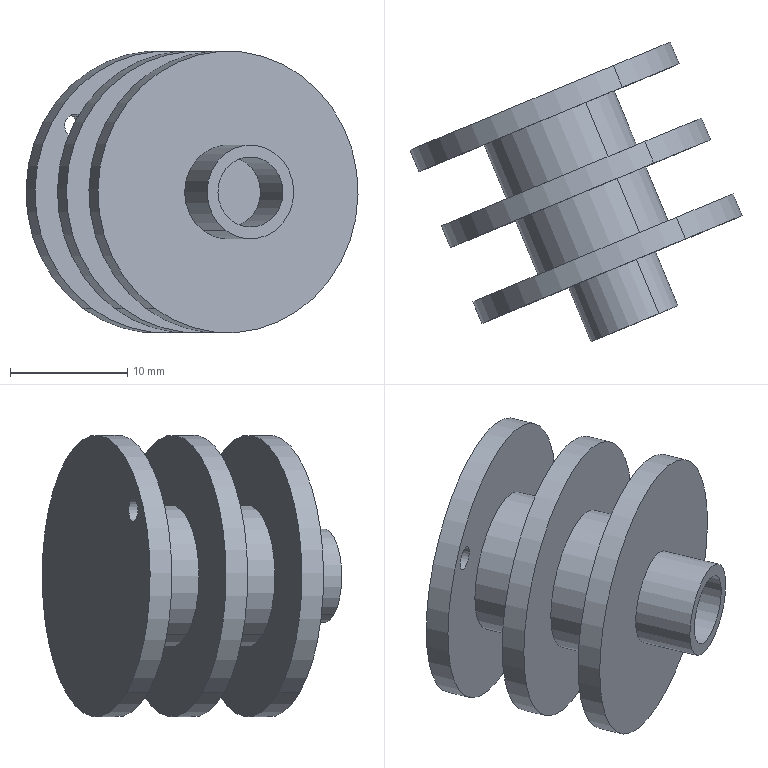Component | SolidWorks | Sensor-1 | 1 solid | 24 faces | box 28.3 x 25.53 x 24 mm | volume 3949 mm3 | cylinder 16 | plane 8 | commonest cylinder face diameters 24 x6 12 x4 2 x2 6 x2 8 x2
build123d program:
from build123d import *

# Parameters (mm, degrees)
SKETCH1_R           = 4
SKETCH1_R_2         = 3
BOSS_EXTRUDE1_DEPTH = 5
SKETCH2_R           = 12
BOSS_EXTRUDE2_DEPTH = 2
SKETCH3_R           = 6
BOSS_EXTRUDE3_DEPTH = 5
SKETCH4_R           = 12
BOSS_EXTRUDE4_DEPTH = 2
SKETCH5_R           = 6
BOSS_EXTRUDE5_DEPTH = 5
SKETCH6_R           = 12
BOSS_EXTRUDE6_DEPTH = 2
SKETCH7_R           = 1
CUT_EXTRUDE1_DEPTH  = 2


with BuildPart() as part:
    # Sketch1 → Boss-Extrude1 (new body)
    with BuildSketch(Plane.XY):
        Circle(SKETCH1_R)
        Circle(SKETCH1_R_2, mode=Mode.SUBTRACT)
    extrude(amount=BOSS_EXTRUDE1_DEPTH)

    # Sketch2 → Boss-Extrude2 (add)
    with BuildSketch(Plane.XY.offset(5)):
        Circle(SKETCH2_R)
    extrude(amount=BOSS_EXTRUDE2_DEPTH)

    # Sketch3 → Boss-Extrude3 (add)
    with BuildSketch(Plane.XY.offset(7)):
        Circle(SKETCH3_R)
    extrude(amount=BOSS_EXTRUDE3_DEPTH)

    # Sketch4 → Boss-Extrude4 (add)
    with BuildSketch(Plane.XY.offset(12)):
        Circle(SKETCH4_R)
    extrude(amount=BOSS_EXTRUDE4_DEPTH)

    # Sketch5 → Boss-Extrude5 (add)
    with BuildSketch(Plane.XY.offset(14)):
        Circle(SKETCH5_R)
    extrude(amount=BOSS_EXTRUDE5_DEPTH)

    # Sketch6 → Boss-Extrude6 (add)
    with BuildSketch(Plane.XY.offset(19)):
        Circle(SKETCH6_R)
    extrude(amount=BOSS_EXTRUDE6_DEPTH)

    # Sketch7 → Cut-Extrude1 (cut)
    with BuildSketch(Plane.XY.offset(21)):
        with Locations((0, 10)):
            Circle(SKETCH7_R)
    extrude(amount=-CUT_EXTRUDE1_DEPTH, mode=Mode.SUBTRACT)


solid = part.part

# Placed as in the assembly
solid = solid.moved(Location((25.514, 19.993, 407.896), (-90, -22.523, 124.32)))
STEP:
#1=COLOUR_RGB('',0.7922,0.8196,0.9333);
#2=FILL_AREA_STYLE_COLOUR('',#1);
#3=FILL_AREA_STYLE('',(#2));
#4=SURFACE_STYLE_FILL_AREA(#3);
#5=SURFACE_SIDE_STYLE('',(#4));
#6=SURFACE_STYLE_USAGE(.BOTH.,#5);
#7=PRESENTATION_STYLE_ASSIGNMENT((#6));
#8=CARTESIAN_POINT('',(0.4381,1.362,16.313));
#9=VERTEX_POINT('',#8);
#10=CARTESIAN_POINT('',(0.3971,1.345,16.248));
#11=VERTEX_POINT('',#10);
#12=CARTESIAN_POINT('',(0.4176,1.354,16.281));
#13=DIRECTION('',(-0.383,0.9237,-0.));
#14=DIRECTION('',(-0.5208,-0.216,-0.8259));
#15=AXIS2_PLACEMENT_3D('',#12,#13,#14);
#16=CIRCLE('',#15,0.03937);
#17=EDGE_CURVE('',#9,#11,#16,.T.);
#18=ORIENTED_EDGE('',*,*,#17,.F.);
#19=CARTESIAN_POINT('',(0.4079,1.435,16.313));
#20=VERTEX_POINT('',#19);
#21=CARTESIAN_POINT('',(0.4381,1.362,16.313));
#22=DIRECTION('',(-0.383,0.9237,-0.));
#23=VECTOR('',#22,39.37);
#24=LINE('',#21,#23);
#25=EDGE_CURVE('',#9,#20,#24,.T.);
#26=ORIENTED_EDGE('',*,*,#25,.T.);
#27=CARTESIAN_POINT('',(0.3669,1.418,16.248));
#28=VERTEX_POINT('',#27);
#29=CARTESIAN_POINT('',(0.3874,1.426,16.281));
#30=DIRECTION('',(-0.383,0.9237,-0.));
#31=DIRECTION('',(-0.5208,-0.216,-0.8259));
#32=AXIS2_PLACEMENT_3D('',#29,#30,#31);
#33=CIRCLE('',#32,0.03937);
#34=EDGE_CURVE('',#20,#28,#33,.T.);
#35=ORIENTED_EDGE('',*,*,#34,.T.);
#36=CARTESIAN_POINT('',(0.3971,1.345,16.248));
#37=DIRECTION('',(-0.383,0.9237,-0.));
#38=VECTOR('',#37,39.37);
#39=LINE('',#36,#38);
#40=EDGE_CURVE('',#11,#28,#39,.T.);
#41=ORIENTED_EDGE('',*,*,#40,.F.);
#42=EDGE_LOOP('',(#18,#26,#35,#41));
#43=FACE_OUTER_BOUND('',#42,.T.);
#44=CARTESIAN_POINT('',(0.4176,1.354,16.281));
#45=DIRECTION('',(-0.383,0.9237,-0.));
#46=DIRECTION('',(-0.5208,-0.216,-0.8259));
#47=AXIS2_PLACEMENT_3D('',#44,#45,#46);
#48=CYLINDRICAL_SURFACE('',#47,0.03937);
#49=ADVANCED_FACE('',(#43),#48,.F.);
#50=CARTESIAN_POINT('',(0.4417,1.449,15.669));
#51=VERTEX_POINT('',#50);
#52=CARTESIAN_POINT('',(0.9338,1.653,16.449));
#53=VERTEX_POINT('',#52);
#54=CARTESIAN_POINT('',(0.6878,1.551,16.059));
#55=DIRECTION('',(-0.383,0.9237,-0.));
#56=DIRECTION('',(-0.5208,-0.216,-0.8259));
#57=AXIS2_PLACEMENT_3D('',#54,#55,#56);
#58=CIRCLE('',#57,0.4724);
#59=EDGE_CURVE('',#51,#53,#58,.T.);
#60=ORIENTED_EDGE('',*,*,#59,.F.);
#61=CARTESIAN_POINT('',(0.4719,1.376,15.669));
#62=VERTEX_POINT('',#61);
#63=CARTESIAN_POINT('',(0.4417,1.449,15.669));
#64=DIRECTION('',(0.383,-0.9237,0.));
#65=VECTOR('',#64,39.37);
#66=LINE('',#63,#65);
#67=EDGE_CURVE('',#51,#62,#66,.T.);
#68=ORIENTED_EDGE('',*,*,#67,.T.);
#69=CARTESIAN_POINT('',(0.964,1.58,16.449));
#70=VERTEX_POINT('',#69);
#71=CARTESIAN_POINT('',(0.7179,1.478,16.059));
#72=DIRECTION('',(-0.383,0.9237,-0.));
#73=DIRECTION('',(-0.5208,-0.216,-0.8259));
#74=AXIS2_PLACEMENT_3D('',#71,#72,#73);
#75=CIRCLE('',#74,0.4724);
#76=EDGE_CURVE('',#62,#70,#75,.T.);
#77=ORIENTED_EDGE('',*,*,#76,.T.);
#78=CARTESIAN_POINT('',(0.9338,1.653,16.449));
#79=DIRECTION('',(0.383,-0.9237,0.));
#80=VECTOR('',#79,39.37);
#81=LINE('',#78,#80);
#82=EDGE_CURVE('',#53,#70,#81,.T.);
#83=ORIENTED_EDGE('',*,*,#82,.F.);
#84=EDGE_LOOP('',(#60,#68,#77,#83));
#85=FACE_OUTER_BOUND('',#84,.T.);
#86=CARTESIAN_POINT('',(0.6878,1.551,16.059));
#87=DIRECTION('',(0.383,-0.9237,0.));
#88=DIRECTION('',(0.5208,0.216,0.8259));
#89=AXIS2_PLACEMENT_3D('',#86,#87,#88);
#90=CYLINDRICAL_SURFACE('',#89,0.4724);
#91=ADVANCED_FACE('',(#85),#90,.T.);
#92=CARTESIAN_POINT('',(0.5949,1.427,15.864));
#93=VERTEX_POINT('',#92);
#94=CARTESIAN_POINT('',(0.841,1.529,16.254));
#95=VERTEX_POINT('',#94);
#96=CARTESIAN_POINT('',(0.7179,1.478,16.059));
#97=DIRECTION('',(-0.383,0.9237,-0.));
#98=DIRECTION('',(-0.5208,-0.216,-0.8259));
#99=AXIS2_PLACEMENT_3D('',#96,#97,#98);
#100=CIRCLE('',#99,0.2362);
#101=EDGE_CURVE('',#93,#95,#100,.T.);
#102=ORIENTED_EDGE('',*,*,#101,.F.);
#103=CARTESIAN_POINT('',(0.6703,1.245,15.864));
#104=VERTEX_POINT('',#103);
#105=CARTESIAN_POINT('',(0.5949,1.427,15.864));
#106=DIRECTION('',(0.383,-0.9237,0.));
#107=VECTOR('',#106,39.37);
#108=LINE('',#105,#107);
#109=EDGE_CURVE('',#93,#104,#108,.T.);
#110=ORIENTED_EDGE('',*,*,#109,.T.);
#111=CARTESIAN_POINT('',(0.9164,1.347,16.254));
#112=VERTEX_POINT('',#111);
#113=CARTESIAN_POINT('',(0.7933,1.296,16.059));
#114=DIRECTION('',(-0.383,0.9237,-0.));
#115=DIRECTION('',(-0.5208,-0.216,-0.8259));
#116=AXIS2_PLACEMENT_3D('',#113,#114,#115);
#117=CIRCLE('',#116,0.2362);
#118=EDGE_CURVE('',#104,#112,#117,.T.);
#119=ORIENTED_EDGE('',*,*,#118,.T.);
#120=CARTESIAN_POINT('',(0.841,1.529,16.254));
#121=DIRECTION('',(0.383,-0.9237,0.));
#122=VECTOR('',#121,39.37);
#123=LINE('',#120,#122);
#124=EDGE_CURVE('',#95,#112,#123,.T.);
#125=ORIENTED_EDGE('',*,*,#124,.F.);
#126=EDGE_LOOP('',(#102,#110,#119,#125));
#127=FACE_OUTER_BOUND('',#126,.T.);
#128=CARTESIAN_POINT('',(0.7179,1.478,16.059));
#129=DIRECTION('',(0.383,-0.9237,0.));
#130=DIRECTION('',(0.5208,0.216,0.8259));
#131=AXIS2_PLACEMENT_3D('',#128,#129,#130);
#132=CYLINDRICAL_SURFACE('',#131,0.2362);
#133=ADVANCED_FACE('',(#127),#132,.T.);
#134=CARTESIAN_POINT('',(0.5473,1.194,15.669));
#135=VERTEX_POINT('',#134);
#136=CARTESIAN_POINT('',(1.039,1.398,16.449));
#137=VERTEX_POINT('',#136);
#138=CARTESIAN_POINT('',(0.7933,1.296,16.059));
#139=DIRECTION('',(-0.383,0.9237,-0.));
#140=DIRECTION('',(-0.5208,-0.216,-0.8259));
#141=AXIS2_PLACEMENT_3D('',#138,#139,#140);
#142=CIRCLE('',#141,0.4724);
#143=EDGE_CURVE('',#135,#137,#142,.T.);
#144=ORIENTED_EDGE('',*,*,#143,.F.);
#145=CARTESIAN_POINT('',(0.5775,1.121,15.669));
#146=VERTEX_POINT('',#145);
#147=CARTESIAN_POINT('',(0.5473,1.194,15.669));
#148=DIRECTION('',(0.383,-0.9237,0.));
#149=VECTOR('',#148,39.37);
#150=LINE('',#147,#149);
#151=EDGE_CURVE('',#135,#146,#150,.T.);
#152=ORIENTED_EDGE('',*,*,#151,.T.);
#153=CARTESIAN_POINT('',(1.07,1.326,16.449));
#154=VERTEX_POINT('',#153);
#155=CARTESIAN_POINT('',(0.8235,1.224,16.059));
#156=DIRECTION('',(-0.383,0.9237,-0.));
#157=DIRECTION('',(-0.5208,-0.216,-0.8259));
#158=AXIS2_PLACEMENT_3D('',#155,#156,#157);
#159=CIRCLE('',#158,0.4724);
#160=EDGE_CURVE('',#146,#154,#159,.T.);
#161=ORIENTED_EDGE('',*,*,#160,.T.);
#162=CARTESIAN_POINT('',(1.039,1.398,16.449));
#163=DIRECTION('',(0.383,-0.9237,0.));
#164=VECTOR('',#163,39.37);
#165=LINE('',#162,#164);
#166=EDGE_CURVE('',#137,#154,#165,.T.);
#167=ORIENTED_EDGE('',*,*,#166,.F.);
#168=EDGE_LOOP('',(#144,#152,#161,#167));
#169=FACE_OUTER_BOUND('',#168,.T.);
#170=CARTESIAN_POINT('',(0.7933,1.296,16.059));
#171=DIRECTION('',(0.383,-0.9237,0.));
#172=DIRECTION('',(0.5208,0.216,0.8259));
#173=AXIS2_PLACEMENT_3D('',#170,#171,#172);
#174=CYLINDRICAL_SURFACE('',#173,0.4724);
#175=ADVANCED_FACE('',(#169),#174,.T.);
#176=CARTESIAN_POINT('',(0.7005,1.173,15.864));
#177=VERTEX_POINT('',#176);
#178=CARTESIAN_POINT('',(0.9465,1.275,16.254));
#179=VERTEX_POINT('',#178);
#180=CARTESIAN_POINT('',(0.8235,1.224,16.059));
#181=DIRECTION('',(-0.383,0.9237,-0.));
#182=DIRECTION('',(-0.5208,-0.216,-0.8259));
#183=AXIS2_PLACEMENT_3D('',#180,#181,#182);
#184=CIRCLE('',#183,0.2362);
#185=EDGE_CURVE('',#177,#179,#184,.T.);
#186=ORIENTED_EDGE('',*,*,#185,.F.);
#187=CARTESIAN_POINT('',(0.7759,0.9907,15.864));
#188=VERTEX_POINT('',#187);
#189=CARTESIAN_POINT('',(0.7005,1.173,15.864));
#190=DIRECTION('',(0.383,-0.9237,0.));
#191=VECTOR('',#190,39.37);
#192=LINE('',#189,#191);
#193=EDGE_CURVE('',#177,#188,#192,.T.);
#194=ORIENTED_EDGE('',*,*,#193,.T.);
#195=CARTESIAN_POINT('',(1.022,1.093,16.254));
#196=VERTEX_POINT('',#195);
#197=CARTESIAN_POINT('',(0.8989,1.042,16.059));
#198=DIRECTION('',(-0.383,0.9237,-0.));
#199=DIRECTION('',(-0.5208,-0.216,-0.8259));
#200=AXIS2_PLACEMENT_3D('',#197,#198,#199);
#201=CIRCLE('',#200,0.2362);
#202=EDGE_CURVE('',#188,#196,#201,.T.);
#203=ORIENTED_EDGE('',*,*,#202,.T.);
#204=CARTESIAN_POINT('',(0.9465,1.275,16.254));
#205=DIRECTION('',(0.383,-0.9237,0.));
#206=VECTOR('',#205,39.37);
#207=LINE('',#204,#206);
#208=EDGE_CURVE('',#179,#196,#207,.T.);
#209=ORIENTED_EDGE('',*,*,#208,.F.);
#210=EDGE_LOOP('',(#186,#194,#203,#209));
#211=FACE_OUTER_BOUND('',#210,.T.);
#212=CARTESIAN_POINT('',(0.8235,1.224,16.059));
#213=DIRECTION('',(0.383,-0.9237,0.));
#214=DIRECTION('',(0.5208,0.216,0.8259));
#215=AXIS2_PLACEMENT_3D('',#212,#213,#214);
#216=CYLINDRICAL_SURFACE('',#215,0.2362);
#217=ADVANCED_FACE('',(#211),#216,.T.);
#218=CARTESIAN_POINT('',(0.6529,0.9397,15.669));
#219=VERTEX_POINT('',#218);
#220=CARTESIAN_POINT('',(1.145,1.144,16.449));
#221=VERTEX_POINT('',#220);
#222=CARTESIAN_POINT('',(0.8989,1.042,16.059));
#223=DIRECTION('',(-0.383,0.9237,-0.));
#224=DIRECTION('',(-0.5208,-0.216,-0.8259));
#225=AXIS2_PLACEMENT_3D('',#222,#223,#224);
#226=CIRCLE('',#225,0.4724);
#227=EDGE_CURVE('',#219,#221,#226,.T.);
#228=ORIENTED_EDGE('',*,*,#227,.F.);
#229=CARTESIAN_POINT('',(0.683,0.8669,15.669));
#230=VERTEX_POINT('',#229);
#231=CARTESIAN_POINT('',(0.6529,0.9397,15.669));
#232=DIRECTION('',(0.383,-0.9237,0.));
#233=VECTOR('',#232,39.37);
#234=LINE('',#231,#233);
#235=EDGE_CURVE('',#219,#230,#234,.T.);
#236=ORIENTED_EDGE('',*,*,#235,.T.);
#237=CARTESIAN_POINT('',(1.175,1.071,16.449));
#238=VERTEX_POINT('',#237);
#239=CARTESIAN_POINT('',(0.9291,0.9689,16.059));
#240=DIRECTION('',(-0.383,0.9237,-0.));
#241=DIRECTION('',(-0.5208,-0.216,-0.8259));
#242=AXIS2_PLACEMENT_3D('',#239,#240,#241);
#243=CIRCLE('',#242,0.4724);
#244=EDGE_CURVE('',#230,#238,#243,.T.);
#245=ORIENTED_EDGE('',*,*,#244,.T.);
#246=CARTESIAN_POINT('',(1.145,1.144,16.449));
#247=DIRECTION('',(0.383,-0.9237,0.));
#248=VECTOR('',#247,39.37);
#249=LINE('',#246,#248);
#250=EDGE_CURVE('',#221,#238,#249,.T.);
#251=ORIENTED_EDGE('',*,*,#250,.F.);
#252=EDGE_LOOP('',(#228,#236,#245,#251));
#253=FACE_OUTER_BOUND('',#252,.T.);
#254=CARTESIAN_POINT('',(0.8989,1.042,16.059));
#255=DIRECTION('',(0.383,-0.9237,0.));
#256=DIRECTION('',(0.5208,0.216,0.8259));
#257=AXIS2_PLACEMENT_3D('',#254,#255,#256);
#258=CYLINDRICAL_SURFACE('',#257,0.4724);
#259=ADVANCED_FACE('',(#253),#258,.T.);
#260=CARTESIAN_POINT('',(0.9906,0.9945,16.156));
#261=VERTEX_POINT('',#260);
#262=CARTESIAN_POINT('',(0.8676,0.9434,15.961));
#263=VERTEX_POINT('',#262);
#264=CARTESIAN_POINT('',(0.9291,0.9689,16.059));
#265=DIRECTION('',(-0.383,0.9237,-0.));
#266=DIRECTION('',(-0.5208,-0.216,-0.8259));
#267=AXIS2_PLACEMENT_3D('',#264,#265,#266);
#268=CIRCLE('',#267,0.1181);
#269=EDGE_CURVE('',#261,#263,#268,.T.);
#270=ORIENTED_EDGE('',*,*,#269,.T.);
#271=CARTESIAN_POINT('',(0.943,0.7616,15.961));
#272=VERTEX_POINT('',#271);
#273=CARTESIAN_POINT('',(0.8676,0.9434,15.961));
#274=DIRECTION('',(0.383,-0.9237,0.));
#275=VECTOR('',#274,39.37);
#276=LINE('',#273,#275);
#277=EDGE_CURVE('',#263,#272,#276,.T.);
#278=ORIENTED_EDGE('',*,*,#277,.T.);
#279=CARTESIAN_POINT('',(1.066,0.8126,16.156));
#280=VERTEX_POINT('',#279);
#281=CARTESIAN_POINT('',(1.004,0.7871,16.059));
#282=DIRECTION('',(-0.383,0.9237,-0.));
#283=DIRECTION('',(-0.5208,-0.216,-0.8259));
#284=AXIS2_PLACEMENT_3D('',#281,#282,#283);
#285=CIRCLE('',#284,0.1181);
#286=EDGE_CURVE('',#280,#272,#285,.T.);
#287=ORIENTED_EDGE('',*,*,#286,.F.);
#288=CARTESIAN_POINT('',(0.9906,0.9945,16.156));
#289=DIRECTION('',(0.383,-0.9237,0.));
#290=VECTOR('',#289,39.37);
#291=LINE('',#288,#290);
#292=EDGE_CURVE('',#261,#280,#291,.T.);
#293=ORIENTED_EDGE('',*,*,#292,.F.);
#294=EDGE_LOOP('',(#270,#278,#287,#293));
#295=FACE_OUTER_BOUND('',#294,.T.);
#296=CARTESIAN_POINT('',(0.9291,0.9689,16.059));
#297=DIRECTION('',(0.383,-0.9237,0.));
#298=DIRECTION('',(0.5208,0.216,0.8259));
#299=AXIS2_PLACEMENT_3D('',#296,#297,#298);
#300=CYLINDRICAL_SURFACE('',#299,0.1181);
#301=ADVANCED_FACE('',(#295),#300,.F.);
#302=CARTESIAN_POINT('',(0.8471,0.9349,15.929));
#303=VERTEX_POINT('',#302);
#304=CARTESIAN_POINT('',(1.011,1.003,16.189));
#305=VERTEX_POINT('',#304);
#306=CARTESIAN_POINT('',(0.9291,0.9689,16.059));
#307=DIRECTION('',(-0.383,0.9237,-0.));
#308=DIRECTION('',(-0.5208,-0.216,-0.8259));
#309=AXIS2_PLACEMENT_3D('',#306,#307,#308);
#310=CIRCLE('',#309,0.1575);
#311=EDGE_CURVE('',#303,#305,#310,.T.);
#312=ORIENTED_EDGE('',*,*,#311,.F.);
#313=CARTESIAN_POINT('',(0.9225,0.7531,15.929));
#314=VERTEX_POINT('',#313);
#315=CARTESIAN_POINT('',(0.8471,0.9349,15.929));
#316=DIRECTION('',(0.383,-0.9237,0.));
#317=VECTOR('',#316,39.37);
#318=LINE('',#315,#317);
#319=EDGE_CURVE('',#303,#314,#318,.T.);
#320=ORIENTED_EDGE('',*,*,#319,.T.);
#321=CARTESIAN_POINT('',(1.086,0.8211,16.189));
#322=VERTEX_POINT('',#321);
#323=CARTESIAN_POINT('',(1.004,0.7871,16.059));
#324=DIRECTION('',(-0.383,0.9237,-0.));
#325=DIRECTION('',(-0.5208,-0.216,-0.8259));
#326=AXIS2_PLACEMENT_3D('',#323,#324,#325);
#327=CIRCLE('',#326,0.1575);
#328=EDGE_CURVE('',#314,#322,#327,.T.);
#329=ORIENTED_EDGE('',*,*,#328,.T.);
#330=CARTESIAN_POINT('',(1.011,1.003,16.189));
#331=DIRECTION('',(0.383,-0.9237,0.));
#332=VECTOR('',#331,39.37);
#333=LINE('',#330,#332);
#334=EDGE_CURVE('',#305,#322,#333,.T.);
#335=ORIENTED_EDGE('',*,*,#334,.F.);
#336=EDGE_LOOP('',(#312,#320,#329,#335));
#337=FACE_OUTER_BOUND('',#336,.T.);
#338=CARTESIAN_POINT('',(0.9291,0.9689,16.059));
#339=DIRECTION('',(0.383,-0.9237,0.));
#340=DIRECTION('',(0.5208,0.216,0.8259));
#341=AXIS2_PLACEMENT_3D('',#338,#339,#340);
#342=CYLINDRICAL_SURFACE('',#341,0.1575);
#343=ADVANCED_FACE('',(#337),#342,.T.);
#344=CARTESIAN_POINT('',(1.004,0.7871,16.059));
#345=DIRECTION('',(-0.383,0.9237,-0.));
#346=DIRECTION('',(-0.5208,-0.216,-0.8259));
#347=AXIS2_PLACEMENT_3D('',#344,#345,#346);
#348=CIRCLE('',#347,0.1575);
#349=EDGE_CURVE('',#322,#314,#348,.T.);
#350=ORIENTED_EDGE('',*,*,#349,.F.);
#351=ORIENTED_EDGE('',*,*,#328,.F.);
#352=EDGE_LOOP('',(#350,#351));
#353=FACE_OUTER_BOUND('',#352,.T.);
#354=ORIENTED_EDGE('',*,*,#286,.T.);
#355=CARTESIAN_POINT('',(1.004,0.7871,16.059));
#356=DIRECTION('',(-0.383,0.9237,-0.));
#357=DIRECTION('',(-0.5208,-0.216,-0.8259));
#358=AXIS2_PLACEMENT_3D('',#355,#356,#357);
#359=CIRCLE('',#358,0.1181);
#360=EDGE_CURVE('',#272,#280,#359,.T.);
#361=ORIENTED_EDGE('',*,*,#360,.T.);
#362=EDGE_LOOP('',(#354,#361));
#363=FACE_BOUND('',#362,.T.);
#364=CARTESIAN_POINT('',(1.004,0.7871,16.059));
#365=DIRECTION('',(-0.383,0.9237,-0.));
#366=DIRECTION('',(-0.5208,-0.216,-0.8259));
#367=AXIS2_PLACEMENT_3D('',#364,#365,#366);
#368=PLANE('',#367);
#369=ADVANCED_FACE('',(#353,#363),#368,.F.);
#370=ORIENTED_EDGE('',*,*,#319,.F.);
#371=CARTESIAN_POINT('',(0.9291,0.9689,16.059));
#372=DIRECTION('',(-0.383,0.9237,-0.));
#373=DIRECTION('',(-0.5208,-0.216,-0.8259));
#374=AXIS2_PLACEMENT_3D('',#371,#372,#373);
#375=CIRCLE('',#374,0.1575);
#376=EDGE_CURVE('',#305,#303,#375,.T.);
#377=ORIENTED_EDGE('',*,*,#376,.F.);
#378=ORIENTED_EDGE('',*,*,#334,.T.);
#379=ORIENTED_EDGE('',*,*,#349,.T.);
#380=EDGE_LOOP('',(#370,#377,#378,#379));
#381=FACE_OUTER_BOUND('',#380,.T.);
#382=CARTESIAN_POINT('',(0.9291,0.9689,16.059));
#383=DIRECTION('',(0.383,-0.9237,0.));
#384=DIRECTION('',(0.5208,0.216,0.8259));
#385=AXIS2_PLACEMENT_3D('',#382,#383,#384);
#386=CYLINDRICAL_SURFACE('',#385,0.1575);
#387=ADVANCED_FACE('',(#381),#386,.T.);
#388=ORIENTED_EDGE('',*,*,#277,.F.);
#389=CARTESIAN_POINT('',(0.9291,0.9689,16.059));
#390=DIRECTION('',(-0.383,0.9237,-0.));
#391=DIRECTION('',(-0.5208,-0.216,-0.8259));
#392=AXIS2_PLACEMENT_3D('',#389,#390,#391);
#393=CIRCLE('',#392,0.1181);
#394=EDGE_CURVE('',#263,#261,#393,.T.);
#395=ORIENTED_EDGE('',*,*,#394,.T.);
#396=ORIENTED_EDGE('',*,*,#292,.T.);
#397=ORIENTED_EDGE('',*,*,#360,.F.);
#398=EDGE_LOOP('',(#388,#395,#396,#397));
#399=FACE_OUTER_BOUND('',#398,.T.);
#400=CARTESIAN_POINT('',(0.9291,0.9689,16.059));
#401=DIRECTION('',(0.383,-0.9237,0.));
#402=DIRECTION('',(0.5208,0.216,0.8259));
#403=AXIS2_PLACEMENT_3D('',#400,#401,#402);
#404=CYLINDRICAL_SURFACE('',#403,0.1181);
#405=ADVANCED_FACE('',(#399),#404,.F.);
#406=ORIENTED_EDGE('',*,*,#269,.F.);
#407=ORIENTED_EDGE('',*,*,#394,.F.);
#408=EDGE_LOOP('',(#406,#407));
#409=FACE_OUTER_BOUND('',#408,.T.);
#410=CARTESIAN_POINT('',(0.9291,0.9689,16.059));
#411=DIRECTION('',(-0.383,0.9237,-0.));
#412=DIRECTION('',(-0.5208,-0.216,-0.8259));
#413=AXIS2_PLACEMENT_3D('',#410,#411,#412);
#414=PLANE('',#413);
#415=ADVANCED_FACE('',(#409),#414,.F.);
#416=ORIENTED_EDGE('',*,*,#235,.F.);
#417=CARTESIAN_POINT('',(0.8989,1.042,16.059));
#418=DIRECTION('',(-0.383,0.9237,-0.));
#419=DIRECTION('',(-0.5208,-0.216,-0.8259));
#420=AXIS2_PLACEMENT_3D('',#417,#418,#419);
#421=CIRCLE('',#420,0.4724);
#422=EDGE_CURVE('',#221,#219,#421,.T.);
#423=ORIENTED_EDGE('',*,*,#422,.F.);
#424=ORIENTED_EDGE('',*,*,#250,.T.);
#425=CARTESIAN_POINT('',(0.9291,0.9689,16.059));
#426=DIRECTION('',(-0.383,0.9237,-0.));
#427=DIRECTION('',(-0.5208,-0.216,-0.8259));
#428=AXIS2_PLACEMENT_3D('',#425,#426,#427);
#429=CIRCLE('',#428,0.4724);
#430=EDGE_CURVE('',#238,#230,#429,.T.);
#431=ORIENTED_EDGE('',*,*,#430,.T.);
#432=EDGE_LOOP('',(#416,#423,#424,#431));
#433=FACE_OUTER_BOUND('',#432,.T.);
#434=CARTESIAN_POINT('',(0.8989,1.042,16.059));
#435=DIRECTION('',(0.383,-0.9237,0.));
#436=DIRECTION('',(0.5208,0.216,0.8259));
#437=AXIS2_PLACEMENT_3D('',#434,#435,#436);
#438=CYLINDRICAL_SURFACE('',#437,0.4724);
#439=ADVANCED_FACE('',(#433),#438,.T.);
#440=CARTESIAN_POINT('',(0.8989,1.042,16.059));
#441=DIRECTION('',(-0.383,0.9237,-0.));
#442=DIRECTION('',(-0.5208,-0.216,-0.8259));
#443=AXIS2_PLACEMENT_3D('',#440,#441,#442);
#444=CIRCLE('',#443,0.2362);
#445=EDGE_CURVE('',#196,#188,#444,.T.);
#446=ORIENTED_EDGE('',*,*,#445,.F.);
#447=ORIENTED_EDGE('',*,*,#202,.F.);
#448=EDGE_LOOP('',(#446,#447));
#449=FACE_BOUND('',#448,.T.);
#450=ORIENTED_EDGE('',*,*,#422,.T.);
#451=ORIENTED_EDGE('',*,*,#227,.T.);
#452=EDGE_LOOP('',(#450,#451));
#453=FACE_OUTER_BOUND('',#452,.T.);
#454=CARTESIAN_POINT('',(0.8989,1.042,16.059));
#455=DIRECTION('',(-0.383,0.9237,-0.));
#456=DIRECTION('',(-0.5208,-0.216,-0.8259));
#457=AXIS2_PLACEMENT_3D('',#454,#455,#456);
#458=PLANE('',#457);
#459=ADVANCED_FACE('',(#449,#453),#458,.T.);
#460=ORIENTED_EDGE('',*,*,#376,.T.);
#461=ORIENTED_EDGE('',*,*,#311,.T.);
#462=EDGE_LOOP('',(#460,#461));
#463=FACE_BOUND('',#462,.T.);
#464=ORIENTED_EDGE('',*,*,#430,.F.);
#465=ORIENTED_EDGE('',*,*,#244,.F.);
#466=EDGE_LOOP('',(#464,#465));
#467=FACE_OUTER_BOUND('',#466,.T.);
#468=CARTESIAN_POINT('',(0.9291,0.9689,16.059));
#469=DIRECTION('',(-0.383,0.9237,-0.));
#470=DIRECTION('',(-0.5208,-0.216,-0.8259));
#471=AXIS2_PLACEMENT_3D('',#468,#469,#470);
#472=PLANE('',#471);
#473=ADVANCED_FACE('',(#463,#467),#472,.F.);
#474=ORIENTED_EDGE('',*,*,#193,.F.);
#475=CARTESIAN_POINT('',(0.8235,1.224,16.059));
#476=DIRECTION('',(-0.383,0.9237,-0.));
#477=DIRECTION('',(-0.5208,-0.216,-0.8259));
#478=AXIS2_PLACEMENT_3D('',#475,#476,#477);
#479=CIRCLE('',#478,0.2362);
#480=EDGE_CURVE('',#179,#177,#479,.T.);
#481=ORIENTED_EDGE('',*,*,#480,.F.);
#482=ORIENTED_EDGE('',*,*,#208,.T.);
#483=ORIENTED_EDGE('',*,*,#445,.T.);
#484=EDGE_LOOP('',(#474,#481,#482,#483));
#485=FACE_OUTER_BOUND('',#484,.T.);
#486=CARTESIAN_POINT('',(0.8235,1.224,16.059));
#487=DIRECTION('',(0.383,-0.9237,0.));
#488=DIRECTION('',(0.5208,0.216,0.8259));
#489=AXIS2_PLACEMENT_3D('',#486,#487,#488);
#490=CYLINDRICAL_SURFACE('',#489,0.2362);
#491=ADVANCED_FACE('',(#485),#490,.T.);
#492=ORIENTED_EDGE('',*,*,#151,.F.);
#493=CARTESIAN_POINT('',(0.7933,1.296,16.059));
#494=DIRECTION('',(-0.383,0.9237,-0.));
#495=DIRECTION('',(-0.5208,-0.216,-0.8259));
#496=AXIS2_PLACEMENT_3D('',#493,#494,#495);
#497=CIRCLE('',#496,0.4724);
#498=EDGE_CURVE('',#137,#135,#497,.T.);
#499=ORIENTED_EDGE('',*,*,#498,.F.);
#500=ORIENTED_EDGE('',*,*,#166,.T.);
#501=CARTESIAN_POINT('',(0.8235,1.224,16.059));
#502=DIRECTION('',(-0.383,0.9237,-0.));
#503=DIRECTION('',(-0.5208,-0.216,-0.8259));
#504=AXIS2_PLACEMENT_3D('',#501,#502,#503);
#505=CIRCLE('',#504,0.4724);
#506=EDGE_CURVE('',#154,#146,#505,.T.);
#507=ORIENTED_EDGE('',*,*,#506,.T.);
#508=EDGE_LOOP('',(#492,#499,#500,#507));
#509=FACE_OUTER_BOUND('',#508,.T.);
#510=CARTESIAN_POINT('',(0.7933,1.296,16.059));
#511=DIRECTION('',(0.383,-0.9237,0.));
#512=DIRECTION('',(0.5208,0.216,0.8259));
#513=AXIS2_PLACEMENT_3D('',#510,#511,#512);
#514=CYLINDRICAL_SURFACE('',#513,0.4724);
#515=ADVANCED_FACE('',(#509),#514,.T.);
#516=CARTESIAN_POINT('',(0.7933,1.296,16.059));
#517=DIRECTION('',(-0.383,0.9237,-0.));
#518=DIRECTION('',(-0.5208,-0.216,-0.8259));
#519=AXIS2_PLACEMENT_3D('',#516,#517,#518);
#520=CIRCLE('',#519,0.2362);
#521=EDGE_CURVE('',#112,#104,#520,.T.);
#522=ORIENTED_EDGE('',*,*,#521,.F.);
#523=ORIENTED_EDGE('',*,*,#118,.F.);
#524=EDGE_LOOP('',(#522,#523));
#525=FACE_BOUND('',#524,.T.);
#526=ORIENTED_EDGE('',*,*,#498,.T.);
#527=ORIENTED_EDGE('',*,*,#143,.T.);
#528=EDGE_LOOP('',(#526,#527));
#529=FACE_OUTER_BOUND('',#528,.T.);
#530=CARTESIAN_POINT('',(0.7933,1.296,16.059));
#531=DIRECTION('',(-0.383,0.9237,-0.));
#532=DIRECTION('',(-0.5208,-0.216,-0.8259));
#533=AXIS2_PLACEMENT_3D('',#530,#531,#532);
#534=PLANE('',#533);
#535=ADVANCED_FACE('',(#525,#529),#534,.T.);
#536=ORIENTED_EDGE('',*,*,#480,.T.);
#537=ORIENTED_EDGE('',*,*,#185,.T.);
#538=EDGE_LOOP('',(#536,#537));
#539=FACE_BOUND('',#538,.T.);
#540=ORIENTED_EDGE('',*,*,#506,.F.);
#541=ORIENTED_EDGE('',*,*,#160,.F.);
#542=EDGE_LOOP('',(#540,#541));
#543=FACE_OUTER_BOUND('',#542,.T.);
#544=CARTESIAN_POINT('',(0.8235,1.224,16.059));
#545=DIRECTION('',(-0.383,0.9237,-0.));
#546=DIRECTION('',(-0.5208,-0.216,-0.8259));
#547=AXIS2_PLACEMENT_3D('',#544,#545,#546);
#548=PLANE('',#547);
#549=ADVANCED_FACE('',(#539,#543),#548,.F.);
#550=ORIENTED_EDGE('',*,*,#109,.F.);
#551=CARTESIAN_POINT('',(0.7179,1.478,16.059));
#552=DIRECTION('',(-0.383,0.9237,-0.));
#553=DIRECTION('',(-0.5208,-0.216,-0.8259));
#554=AXIS2_PLACEMENT_3D('',#551,#552,#553);
#555=CIRCLE('',#554,0.2362);
#556=EDGE_CURVE('',#95,#93,#555,.T.);
#557=ORIENTED_EDGE('',*,*,#556,.F.);
#558=ORIENTED_EDGE('',*,*,#124,.T.);
#559=ORIENTED_EDGE('',*,*,#521,.T.);
#560=EDGE_LOOP('',(#550,#557,#558,#559));
#561=FACE_OUTER_BOUND('',#560,.T.);
#562=CARTESIAN_POINT('',(0.7179,1.478,16.059));
#563=DIRECTION('',(0.383,-0.9237,0.));
#564=DIRECTION('',(0.5208,0.216,0.8259));
#565=AXIS2_PLACEMENT_3D('',#562,#563,#564);
#566=CYLINDRICAL_SURFACE('',#565,0.2362);
#567=ADVANCED_FACE('',(#561),#566,.T.);
#568=ORIENTED_EDGE('',*,*,#67,.F.);
#569=CARTESIAN_POINT('',(0.6878,1.551,16.059));
#570=DIRECTION('',(-0.383,0.9237,-0.));
#571=DIRECTION('',(-0.5208,-0.216,-0.8259));
#572=AXIS2_PLACEMENT_3D('',#569,#570,#571);
#573=CIRCLE('',#572,0.4724);
#574=EDGE_CURVE('',#53,#51,#573,.T.);
#575=ORIENTED_EDGE('',*,*,#574,.F.);
#576=ORIENTED_EDGE('',*,*,#82,.T.);
#577=CARTESIAN_POINT('',(0.7179,1.478,16.059));
#578=DIRECTION('',(-0.383,0.9237,-0.));
#579=DIRECTION('',(-0.5208,-0.216,-0.8259));
#580=AXIS2_PLACEMENT_3D('',#577,#578,#579);
#581=CIRCLE('',#580,0.4724);
#582=EDGE_CURVE('',#70,#62,#581,.T.);
#583=ORIENTED_EDGE('',*,*,#582,.T.);
#584=EDGE_LOOP('',(#568,#575,#576,#583));
#585=FACE_OUTER_BOUND('',#584,.T.);
#586=CARTESIAN_POINT('',(0.6878,1.551,16.059));
#587=DIRECTION('',(0.383,-0.9237,0.));
#588=DIRECTION('',(0.5208,0.216,0.8259));
#589=AXIS2_PLACEMENT_3D('',#586,#587,#588);
#590=CYLINDRICAL_SURFACE('',#589,0.4724);
#591=ADVANCED_FACE('',(#585),#590,.T.);
#592=CARTESIAN_POINT('',(0.3874,1.426,16.281));
#593=DIRECTION('',(-0.383,0.9237,-0.));
#594=DIRECTION('',(-0.5208,-0.216,-0.8259));
#595=AXIS2_PLACEMENT_3D('',#592,#593,#594);
#596=CIRCLE('',#595,0.03937);
#597=EDGE_CURVE('',#28,#20,#596,.T.);
#598=ORIENTED_EDGE('',*,*,#597,.F.);
#599=ORIENTED_EDGE('',*,*,#34,.F.);
#600=EDGE_LOOP('',(#598,#599));
#601=FACE_BOUND('',#600,.T.);
#602=ORIENTED_EDGE('',*,*,#574,.T.);
#603=ORIENTED_EDGE('',*,*,#59,.T.);
#604=EDGE_LOOP('',(#602,#603));
#605=FACE_OUTER_BOUND('',#604,.T.);
#606=CARTESIAN_POINT('',(0.6878,1.551,16.059));
#607=DIRECTION('',(-0.383,0.9237,-0.));
#608=DIRECTION('',(-0.5208,-0.216,-0.8259));
#609=AXIS2_PLACEMENT_3D('',#606,#607,#608);
#610=PLANE('',#609);
#611=ADVANCED_FACE('',(#601,#605),#610,.T.);
#612=CARTESIAN_POINT('',(0.4176,1.354,16.281));
#613=DIRECTION('',(-0.383,0.9237,-0.));
#614=DIRECTION('',(-0.5208,-0.216,-0.8259));
#615=AXIS2_PLACEMENT_3D('',#612,#613,#614);
#616=CIRCLE('',#615,0.03937);
#617=EDGE_CURVE('',#11,#9,#616,.T.);
#618=ORIENTED_EDGE('',*,*,#617,.T.);
#619=ORIENTED_EDGE('',*,*,#17,.T.);
#620=EDGE_LOOP('',(#618,#619));
#621=FACE_BOUND('',#620,.T.);
#622=ORIENTED_EDGE('',*,*,#556,.T.);
#623=ORIENTED_EDGE('',*,*,#101,.T.);
#624=EDGE_LOOP('',(#622,#623));
#625=FACE_BOUND('',#624,.T.);
#626=ORIENTED_EDGE('',*,*,#582,.F.);
#627=ORIENTED_EDGE('',*,*,#76,.F.);
#628=EDGE_LOOP('',(#626,#627));
#629=FACE_OUTER_BOUND('',#628,.T.);
#630=CARTESIAN_POINT('',(0.7179,1.478,16.059));
#631=DIRECTION('',(-0.383,0.9237,-0.));
#632=DIRECTION('',(-0.5208,-0.216,-0.8259));
#633=AXIS2_PLACEMENT_3D('',#630,#631,#632);
#634=PLANE('',#633);
#635=ADVANCED_FACE('',(#621,#625,#629),#634,.F.);
#636=ORIENTED_EDGE('',*,*,#25,.F.);
#637=ORIENTED_EDGE('',*,*,#617,.F.);
#638=ORIENTED_EDGE('',*,*,#40,.T.);
#639=ORIENTED_EDGE('',*,*,#597,.T.);
#640=EDGE_LOOP('',(#636,#637,#638,#639));
#641=FACE_OUTER_BOUND('',#640,.T.);
#642=CARTESIAN_POINT('',(0.4176,1.354,16.281));
#643=DIRECTION('',(-0.383,0.9237,-0.));
#644=DIRECTION('',(-0.5208,-0.216,-0.8259));
#645=AXIS2_PLACEMENT_3D('',#642,#643,#644);
#646=CYLINDRICAL_SURFACE('',#645,0.03937);
#647=ADVANCED_FACE('',(#641),#646,.F.);
#648=CLOSED_SHELL('',(#49,#91,#133,#175,#217,#259,#301,#343,#369,#387,#405,#415,#439,#459,#473,#491,#515,#535,#549,#567,#591,#611,#635,#647));
#649=MANIFOLD_SOLID_BREP('',#648);
#650=STYLED_ITEM('',(#7),#649);
#651=(LENGTH_UNIT()NAMED_UNIT(*)SI_UNIT($,.METRE.));
#652=LENGTH_MEASURE_WITH_UNIT(LENGTH_MEASURE(0.0254),#651);
#653=DIMENSIONAL_EXPONENTS(1.,0.,0.,0.,0.,0.,0.);
#654=(CONVERSION_BASED_UNIT('',#652)LENGTH_UNIT()NAMED_UNIT(#653));
#655=UNCERTAINTY_MEASURE_WITH_UNIT(LENGTH_MEASURE(0.00001),#654,'','');
#656=(NAMED_UNIT(*)PLANE_ANGLE_UNIT()SI_UNIT($,.RADIAN.));
#657=(NAMED_UNIT(*)SI_UNIT($,.STERADIAN.)SOLID_ANGLE_UNIT());
#658=(GEOMETRIC_REPRESENTATION_CONTEXT(3)GLOBAL_UNCERTAINTY_ASSIGNED_CONTEXT((#655))GLOBAL_UNIT_ASSIGNED_CONTEXT((#654,#656,#657))REPRESENTATION_CONTEXT('',''));
#659=MECHANICAL_DESIGN_GEOMETRIC_PRESENTATION_REPRESENTATION('',(#650),#658);
#660=PRESENTATION_LAYER_ASSIGNMENT('','',(#650));
#661=CARTESIAN_POINT('',(0.,0.,0.));
#662=DIRECTION('',(0.,0.,1.));
#663=DIRECTION('',(1.,0.,0.));
#664=AXIS2_PLACEMENT_3D('',#661,#662,#663);
#665=(LENGTH_UNIT()NAMED_UNIT(*)SI_UNIT($,.METRE.));
#666=LENGTH_MEASURE_WITH_UNIT(LENGTH_MEASURE(0.0254),#665);
#667=DIMENSIONAL_EXPONENTS(1.,0.,0.,0.,0.,0.,0.);
#668=(CONVERSION_BASED_UNIT('',#666)LENGTH_UNIT()NAMED_UNIT(#667));
#669=UNCERTAINTY_MEASURE_WITH_UNIT(LENGTH_MEASURE(0.00001),#668,'','');
#670=(NAMED_UNIT(*)PLANE_ANGLE_UNIT()SI_UNIT($,.RADIAN.));
#671=(NAMED_UNIT(*)SI_UNIT($,.STERADIAN.)SOLID_ANGLE_UNIT());
#672=(GEOMETRIC_REPRESENTATION_CONTEXT(3)GLOBAL_UNCERTAINTY_ASSIGNED_CONTEXT((#669))GLOBAL_UNIT_ASSIGNED_CONTEXT((#668,#670,#671))REPRESENTATION_CONTEXT('',''));
#673=ADVANCED_BREP_SHAPE_REPRESENTATION('',(#649,#664),#672);